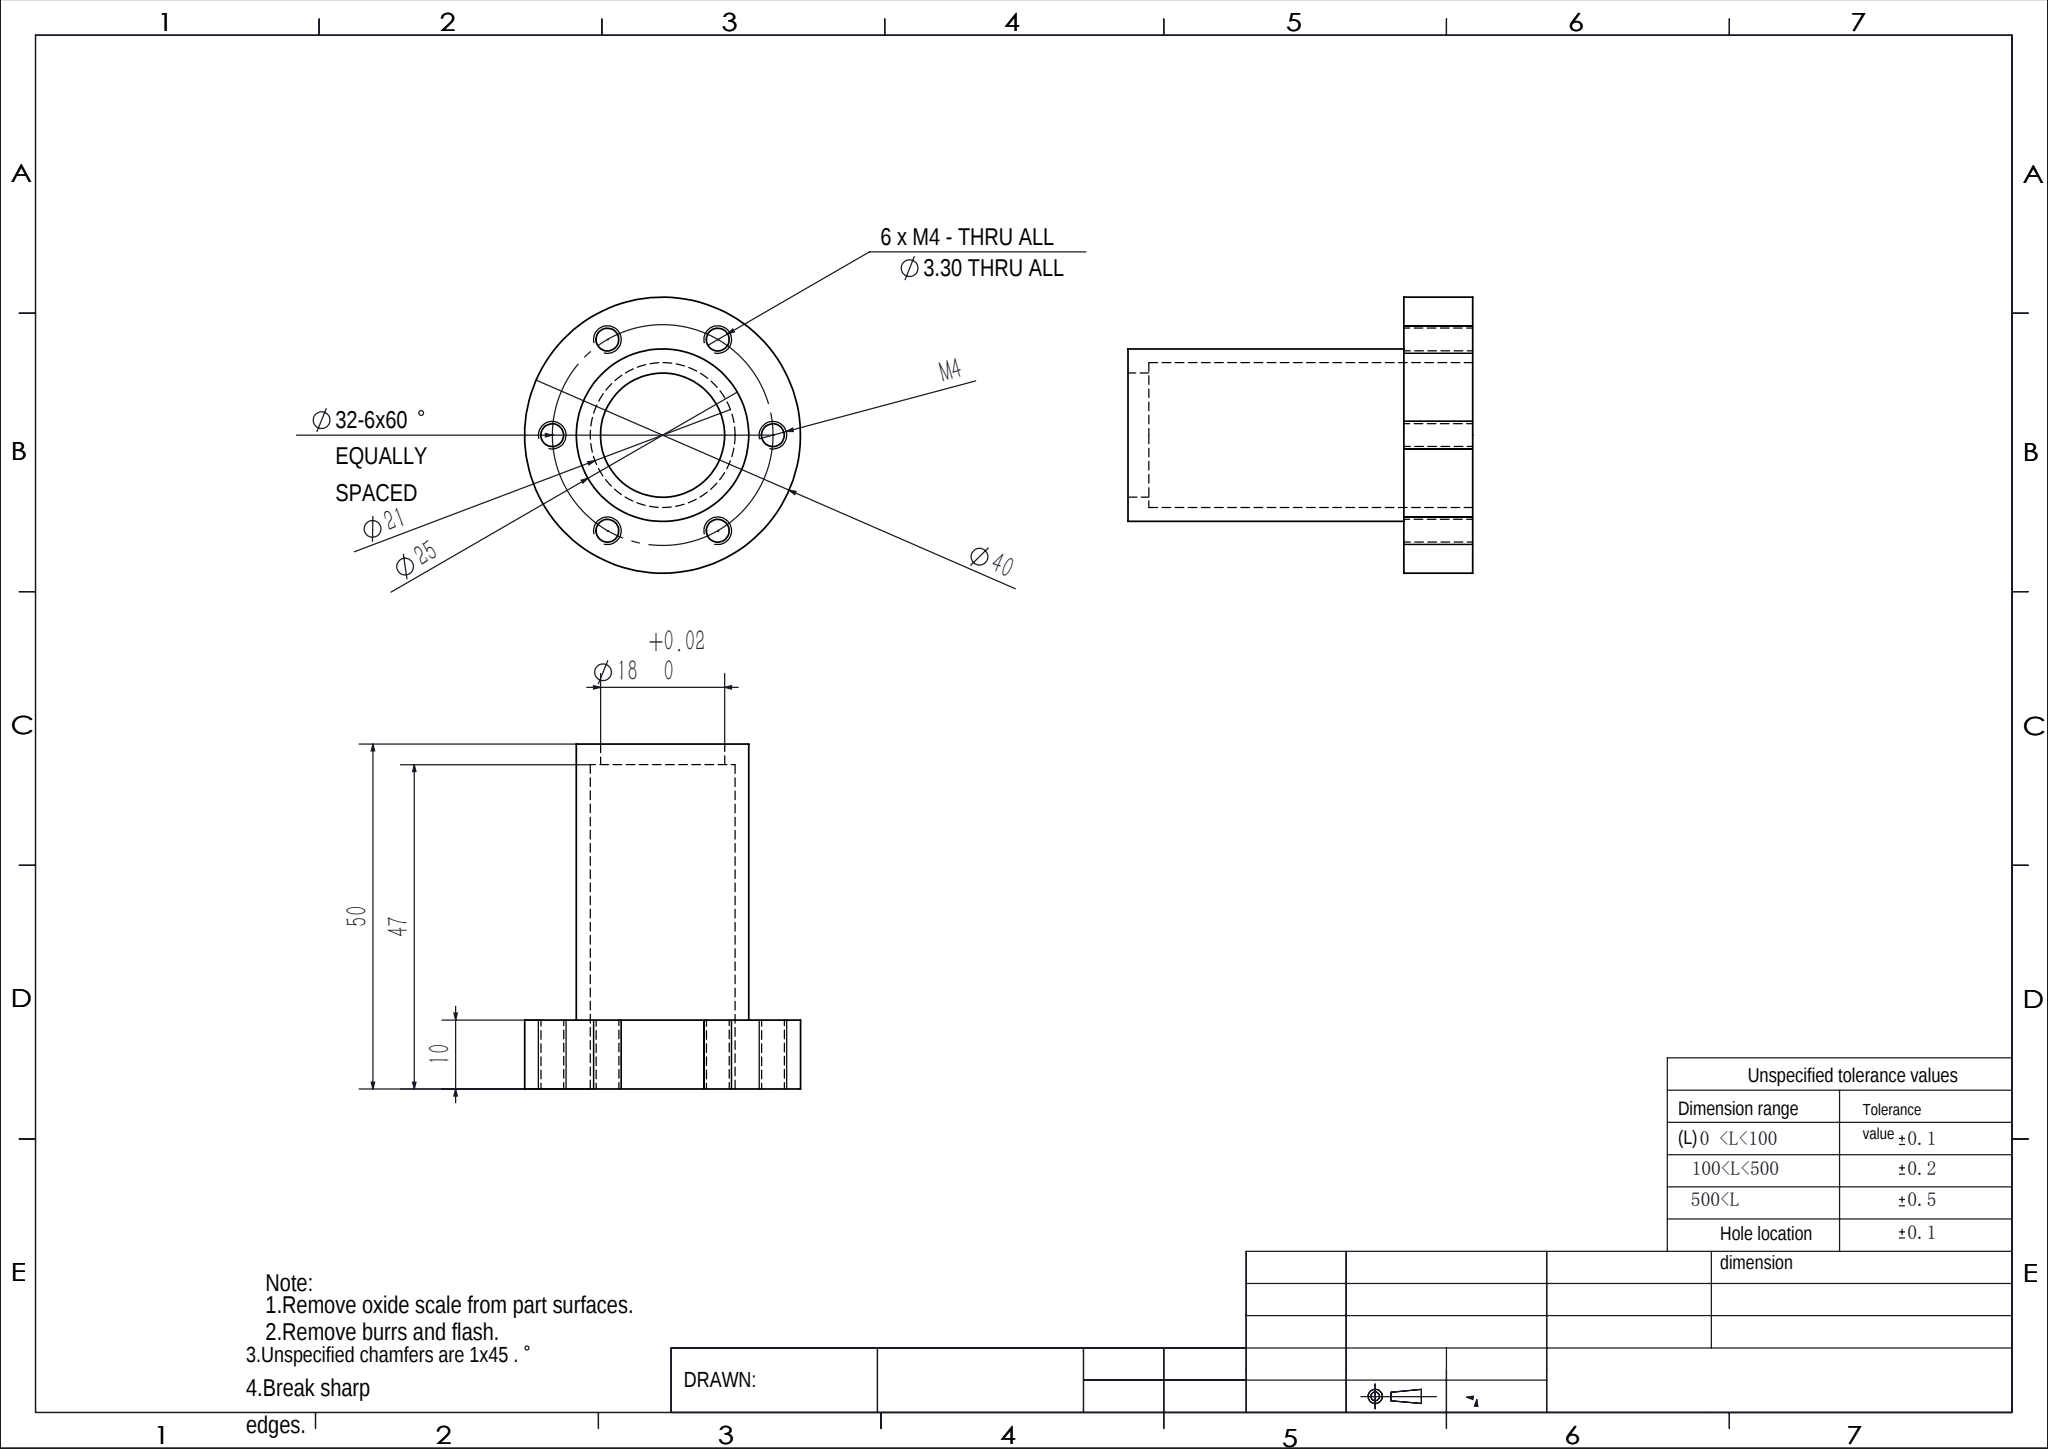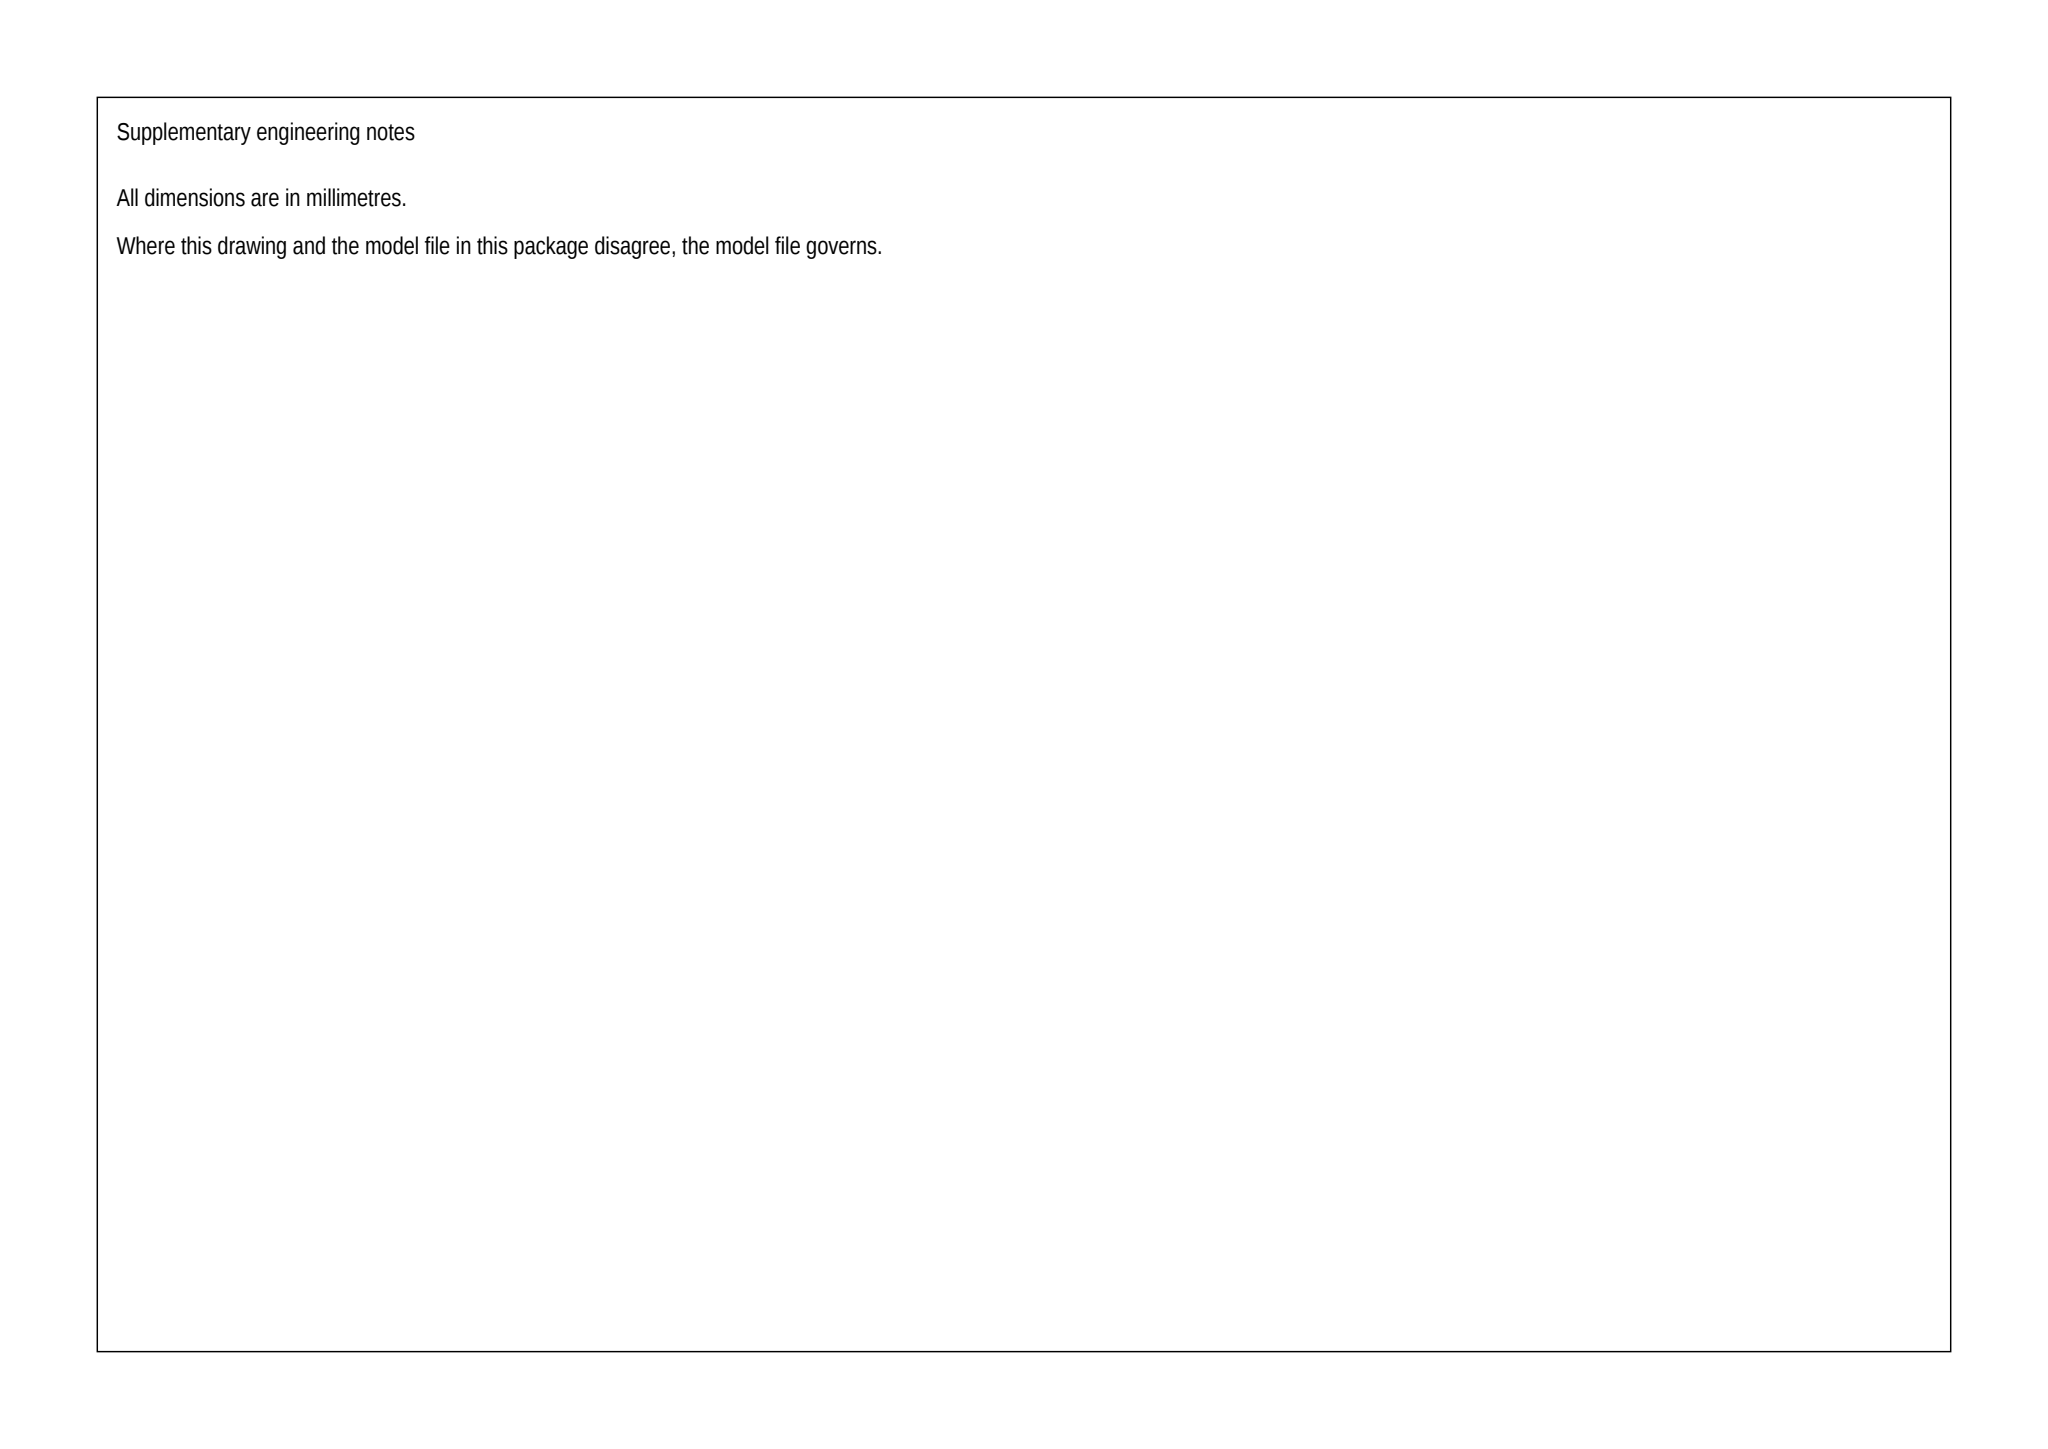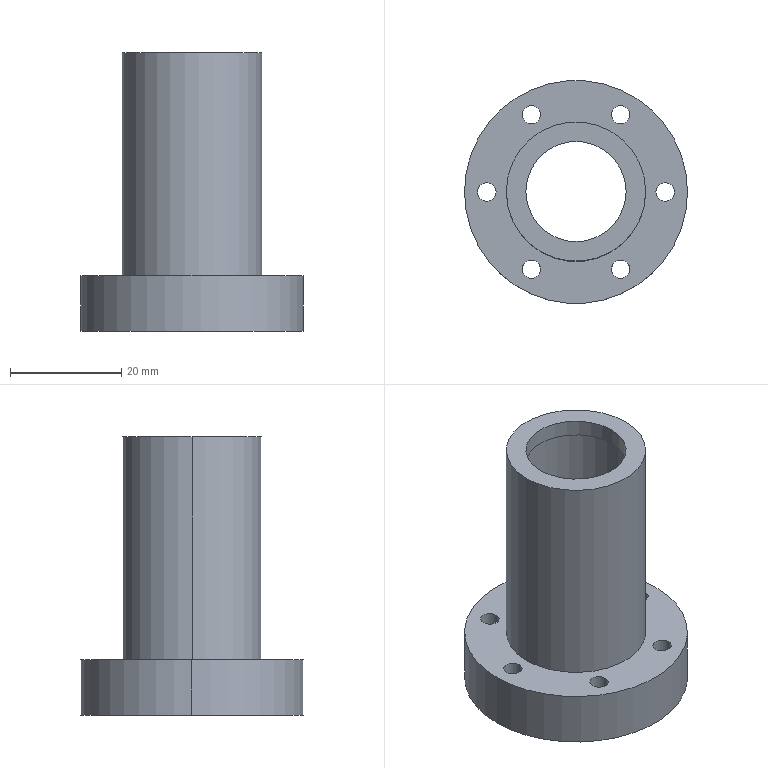Part | SolidWorks | mm | material 6061 | 1 solid | 24 faces | box 40 x 40 x 50 mm | volume 14646 mm3 | cylinder 20 | plane 4 | commonest cylinder face diameters 3.3 x12 25 x2 18 x2 40 x2 21 x2
Drawing notes:
UNSPECIFIED CHAMFERS 1 x 45 DEG; BLUNT SHARP CORNERS | from the solid: No inclined_planes/cones in STEP; garbled "1x454" = 1x45 deg chamfer note only
build123d program:
from build123d import *

# Parameters (mm, degrees)
SKETCH1_R           = 20
BOSS_EXTRUDE1_DEPTH = 50
SKETCH2_R           = 10.5
CUT_EXTRUDE1_DEPTH  = 58.446
BOSS_EXTRUDE2_START = -3
SKETCH3_R           = 10.5
SKETCH3_R_2         = 9
BOSS_EXTRUDE2_DEPTH = 3
CUT_EXTRUDE2_START  = -10
SKETCH4_R           = 23.5
SKETCH4_R_2         = 12.5
CUT_EXTRUDE2_DEPTH  = 48.446
M4_TAPPED_HOLE1_D   = 3.3


with BuildPart() as part:
    # Sketch1 → Boss-Extrude1 (new body)
    with BuildSketch(Plane.XY):
        Circle(SKETCH1_R)
    extrude(amount=BOSS_EXTRUDE1_DEPTH)

    # Sketch2 → Cut-Extrude1 (cut, through all)
    with BuildSketch(Plane(origin=(0, 0, 0), x_dir=(-1, 0, 0), z_dir=(0, 0, -1))):
        Circle(SKETCH2_R)
    extrude(amount=-CUT_EXTRUDE1_DEPTH, mode=Mode.SUBTRACT)

    # Sketch3 → Boss-Extrude2 (add)
    with BuildSketch(Plane.XY.offset(50).offset(BOSS_EXTRUDE2_START)):
        with Locations(Location((0, 0, 0), (0, 0, 180))):
            Circle(SKETCH3_R)
        Circle(SKETCH3_R_2, mode=Mode.SUBTRACT)
    extrude(amount=BOSS_EXTRUDE2_DEPTH)

    # Sketch4 → Cut-Extrude2 (cut, through all)
    with BuildSketch(Plane(origin=(0, 0, 0), x_dir=(-1, 0, 0), z_dir=(0, 0, -1)).offset(CUT_EXTRUDE2_START)):
        Circle(SKETCH4_R)
        Circle(SKETCH4_R_2, mode=Mode.SUBTRACT)
    extrude(amount=-CUT_EXTRUDE2_DEPTH, mode=Mode.SUBTRACT)

    # M4 Tapped Hole1 (through all)
    with Locations(Plane(origin=(0, 0, 0), x_dir=(-1, 0, 0), z_dir=(0, 0, -1))):
        with Locations((-16, 0), (-8, 13.856), (8, 13.856), (16, 0), (8, -13.856), (-8, -13.856), (0, 0)):
            Hole(M4_TAPPED_HOLE1_D / 2)


solid = part.part
STEP:
#1=CARTESIAN_POINT('',(17.65,0.,10.));
#2=VERTEX_POINT('',#1);
#3=CARTESIAN_POINT('',(14.35,0.,10.));
#4=VERTEX_POINT('',#3);
#5=CARTESIAN_POINT('',(16.,0.,10.));
#6=DIRECTION('',(0.,0.,-1.));
#7=DIRECTION('',(-1.,0.,0.));
#8=AXIS2_PLACEMENT_3D('',#5,#6,#7);
#9=CIRCLE('',#8,1.65);
#10=EDGE_CURVE('',#2,#4,#9,.T.);
#11=ORIENTED_EDGE('',*,*,#10,.F.);
#12=CARTESIAN_POINT('',(17.65,0.,-0.));
#13=VERTEX_POINT('',#12);
#14=CARTESIAN_POINT('',(17.65,0.,0.));
#15=DIRECTION('',(0.,0.,-1.));
#16=VECTOR('',#15,1000.);
#17=LINE('',#14,#16);
#18=EDGE_CURVE('',#2,#13,#17,.T.);
#19=ORIENTED_EDGE('',*,*,#18,.T.);
#20=CARTESIAN_POINT('',(14.35,0.,-0.));
#21=VERTEX_POINT('',#20);
#22=CARTESIAN_POINT('',(16.,0.,-0.));
#23=DIRECTION('',(0.,0.,-1.));
#24=DIRECTION('',(-1.,0.,0.));
#25=AXIS2_PLACEMENT_3D('',#22,#23,#24);
#26=CIRCLE('',#25,1.65);
#27=EDGE_CURVE('',#13,#21,#26,.T.);
#28=ORIENTED_EDGE('',*,*,#27,.T.);
#29=CARTESIAN_POINT('',(14.35,0.,0.));
#30=DIRECTION('',(0.,0.,-1.));
#31=VECTOR('',#30,1000.);
#32=LINE('',#29,#31);
#33=EDGE_CURVE('',#4,#21,#32,.T.);
#34=ORIENTED_EDGE('',*,*,#33,.F.);
#35=EDGE_LOOP('',(#11,#19,#28,#34));
#36=FACE_OUTER_BOUND('',#35,.T.);
#37=CARTESIAN_POINT('',(16.,0.,0.));
#38=DIRECTION('',(0.,0.,-1.));
#39=DIRECTION('',(-1.,0.,0.));
#40=AXIS2_PLACEMENT_3D('',#37,#38,#39);
#41=CYLINDRICAL_SURFACE('',#40,1.65);
#42=ADVANCED_FACE('',(#36),#41,.F.);
#43=CARTESIAN_POINT('',(9.65,13.856,10.));
#44=VERTEX_POINT('',#43);
#45=CARTESIAN_POINT('',(6.35,13.856,10.));
#46=VERTEX_POINT('',#45);
#47=CARTESIAN_POINT('',(8.,13.856,10.));
#48=DIRECTION('',(0.,0.,-1.));
#49=DIRECTION('',(-1.,0.,0.));
#50=AXIS2_PLACEMENT_3D('',#47,#48,#49);
#51=CIRCLE('',#50,1.65);
#52=EDGE_CURVE('',#44,#46,#51,.T.);
#53=ORIENTED_EDGE('',*,*,#52,.F.);
#54=CARTESIAN_POINT('',(9.65,13.856,-0.));
#55=VERTEX_POINT('',#54);
#56=CARTESIAN_POINT('',(9.65,13.856,0.));
#57=DIRECTION('',(0.,0.,-1.));
#58=VECTOR('',#57,1000.);
#59=LINE('',#56,#58);
#60=EDGE_CURVE('',#44,#55,#59,.T.);
#61=ORIENTED_EDGE('',*,*,#60,.T.);
#62=CARTESIAN_POINT('',(6.35,13.856,-0.));
#63=VERTEX_POINT('',#62);
#64=CARTESIAN_POINT('',(8.,13.856,-0.));
#65=DIRECTION('',(0.,0.,-1.));
#66=DIRECTION('',(-1.,0.,0.));
#67=AXIS2_PLACEMENT_3D('',#64,#65,#66);
#68=CIRCLE('',#67,1.65);
#69=EDGE_CURVE('',#55,#63,#68,.T.);
#70=ORIENTED_EDGE('',*,*,#69,.T.);
#71=CARTESIAN_POINT('',(6.35,13.856,0.));
#72=DIRECTION('',(0.,0.,-1.));
#73=VECTOR('',#72,1000.);
#74=LINE('',#71,#73);
#75=EDGE_CURVE('',#46,#63,#74,.T.);
#76=ORIENTED_EDGE('',*,*,#75,.F.);
#77=EDGE_LOOP('',(#53,#61,#70,#76));
#78=FACE_OUTER_BOUND('',#77,.T.);
#79=CARTESIAN_POINT('',(8.,13.856,0.));
#80=DIRECTION('',(0.,0.,-1.));
#81=DIRECTION('',(-1.,0.,0.));
#82=AXIS2_PLACEMENT_3D('',#79,#80,#81);
#83=CYLINDRICAL_SURFACE('',#82,1.65);
#84=ADVANCED_FACE('',(#78),#83,.F.);
#85=CARTESIAN_POINT('',(-6.35,13.856,10.));
#86=VERTEX_POINT('',#85);
#87=CARTESIAN_POINT('',(-9.65,13.856,10.));
#88=VERTEX_POINT('',#87);
#89=CARTESIAN_POINT('',(-8.,13.856,10.));
#90=DIRECTION('',(0.,0.,-1.));
#91=DIRECTION('',(-1.,0.,0.));
#92=AXIS2_PLACEMENT_3D('',#89,#90,#91);
#93=CIRCLE('',#92,1.65);
#94=EDGE_CURVE('',#86,#88,#93,.T.);
#95=ORIENTED_EDGE('',*,*,#94,.F.);
#96=CARTESIAN_POINT('',(-6.35,13.856,-0.));
#97=VERTEX_POINT('',#96);
#98=CARTESIAN_POINT('',(-6.35,13.856,0.));
#99=DIRECTION('',(0.,0.,-1.));
#100=VECTOR('',#99,1000.);
#101=LINE('',#98,#100);
#102=EDGE_CURVE('',#86,#97,#101,.T.);
#103=ORIENTED_EDGE('',*,*,#102,.T.);
#104=CARTESIAN_POINT('',(-9.65,13.856,-0.));
#105=VERTEX_POINT('',#104);
#106=CARTESIAN_POINT('',(-8.,13.856,-0.));
#107=DIRECTION('',(0.,0.,-1.));
#108=DIRECTION('',(-1.,0.,0.));
#109=AXIS2_PLACEMENT_3D('',#106,#107,#108);
#110=CIRCLE('',#109,1.65);
#111=EDGE_CURVE('',#97,#105,#110,.T.);
#112=ORIENTED_EDGE('',*,*,#111,.T.);
#113=CARTESIAN_POINT('',(-9.65,13.856,0.));
#114=DIRECTION('',(0.,0.,-1.));
#115=VECTOR('',#114,1000.);
#116=LINE('',#113,#115);
#117=EDGE_CURVE('',#88,#105,#116,.T.);
#118=ORIENTED_EDGE('',*,*,#117,.F.);
#119=EDGE_LOOP('',(#95,#103,#112,#118));
#120=FACE_OUTER_BOUND('',#119,.T.);
#121=CARTESIAN_POINT('',(-8.,13.856,0.));
#122=DIRECTION('',(0.,0.,-1.));
#123=DIRECTION('',(-1.,0.,0.));
#124=AXIS2_PLACEMENT_3D('',#121,#122,#123);
#125=CYLINDRICAL_SURFACE('',#124,1.65);
#126=ADVANCED_FACE('',(#120),#125,.F.);
#127=CARTESIAN_POINT('',(-14.35,-0.,10.));
#128=VERTEX_POINT('',#127);
#129=CARTESIAN_POINT('',(-17.65,-0.,10.));
#130=VERTEX_POINT('',#129);
#131=CARTESIAN_POINT('',(-16.,-0.,10.));
#132=DIRECTION('',(0.,0.,-1.));
#133=DIRECTION('',(-1.,0.,0.));
#134=AXIS2_PLACEMENT_3D('',#131,#132,#133);
#135=CIRCLE('',#134,1.65);
#136=EDGE_CURVE('',#128,#130,#135,.T.);
#137=ORIENTED_EDGE('',*,*,#136,.F.);
#138=CARTESIAN_POINT('',(-14.35,-0.,-0.));
#139=VERTEX_POINT('',#138);
#140=CARTESIAN_POINT('',(-14.35,-0.,0.));
#141=DIRECTION('',(0.,0.,-1.));
#142=VECTOR('',#141,1000.);
#143=LINE('',#140,#142);
#144=EDGE_CURVE('',#128,#139,#143,.T.);
#145=ORIENTED_EDGE('',*,*,#144,.T.);
#146=CARTESIAN_POINT('',(-17.65,-0.,-0.));
#147=VERTEX_POINT('',#146);
#148=CARTESIAN_POINT('',(-16.,-0.,-0.));
#149=DIRECTION('',(0.,0.,-1.));
#150=DIRECTION('',(-1.,0.,0.));
#151=AXIS2_PLACEMENT_3D('',#148,#149,#150);
#152=CIRCLE('',#151,1.65);
#153=EDGE_CURVE('',#139,#147,#152,.T.);
#154=ORIENTED_EDGE('',*,*,#153,.T.);
#155=CARTESIAN_POINT('',(-17.65,-0.,0.));
#156=DIRECTION('',(0.,0.,-1.));
#157=VECTOR('',#156,1000.);
#158=LINE('',#155,#157);
#159=EDGE_CURVE('',#130,#147,#158,.T.);
#160=ORIENTED_EDGE('',*,*,#159,.F.);
#161=EDGE_LOOP('',(#137,#145,#154,#160));
#162=FACE_OUTER_BOUND('',#161,.T.);
#163=CARTESIAN_POINT('',(-16.,-0.,0.));
#164=DIRECTION('',(0.,0.,-1.));
#165=DIRECTION('',(-1.,0.,0.));
#166=AXIS2_PLACEMENT_3D('',#163,#164,#165);
#167=CYLINDRICAL_SURFACE('',#166,1.65);
#168=ADVANCED_FACE('',(#162),#167,.F.);
#169=CARTESIAN_POINT('',(-6.35,-13.856,10.));
#170=VERTEX_POINT('',#169);
#171=CARTESIAN_POINT('',(-9.65,-13.856,10.));
#172=VERTEX_POINT('',#171);
#173=CARTESIAN_POINT('',(-8.,-13.856,10.));
#174=DIRECTION('',(0.,0.,-1.));
#175=DIRECTION('',(-1.,0.,0.));
#176=AXIS2_PLACEMENT_3D('',#173,#174,#175);
#177=CIRCLE('',#176,1.65);
#178=EDGE_CURVE('',#170,#172,#177,.T.);
#179=ORIENTED_EDGE('',*,*,#178,.F.);
#180=CARTESIAN_POINT('',(-6.35,-13.856,-0.));
#181=VERTEX_POINT('',#180);
#182=CARTESIAN_POINT('',(-6.35,-13.856,0.));
#183=DIRECTION('',(0.,0.,-1.));
#184=VECTOR('',#183,1000.);
#185=LINE('',#182,#184);
#186=EDGE_CURVE('',#170,#181,#185,.T.);
#187=ORIENTED_EDGE('',*,*,#186,.T.);
#188=CARTESIAN_POINT('',(-9.65,-13.856,-0.));
#189=VERTEX_POINT('',#188);
#190=CARTESIAN_POINT('',(-8.,-13.856,-0.));
#191=DIRECTION('',(0.,0.,-1.));
#192=DIRECTION('',(-1.,0.,0.));
#193=AXIS2_PLACEMENT_3D('',#190,#191,#192);
#194=CIRCLE('',#193,1.65);
#195=EDGE_CURVE('',#181,#189,#194,.T.);
#196=ORIENTED_EDGE('',*,*,#195,.T.);
#197=CARTESIAN_POINT('',(-9.65,-13.856,0.));
#198=DIRECTION('',(0.,0.,-1.));
#199=VECTOR('',#198,1000.);
#200=LINE('',#197,#199);
#201=EDGE_CURVE('',#172,#189,#200,.T.);
#202=ORIENTED_EDGE('',*,*,#201,.F.);
#203=EDGE_LOOP('',(#179,#187,#196,#202));
#204=FACE_OUTER_BOUND('',#203,.T.);
#205=CARTESIAN_POINT('',(-8.,-13.856,0.));
#206=DIRECTION('',(0.,0.,-1.));
#207=DIRECTION('',(-1.,0.,0.));
#208=AXIS2_PLACEMENT_3D('',#205,#206,#207);
#209=CYLINDRICAL_SURFACE('',#208,1.65);
#210=ADVANCED_FACE('',(#204),#209,.F.);
#211=CARTESIAN_POINT('',(9.65,-13.856,10.));
#212=VERTEX_POINT('',#211);
#213=CARTESIAN_POINT('',(6.35,-13.856,10.));
#214=VERTEX_POINT('',#213);
#215=CARTESIAN_POINT('',(8.,-13.856,10.));
#216=DIRECTION('',(0.,0.,-1.));
#217=DIRECTION('',(-1.,0.,0.));
#218=AXIS2_PLACEMENT_3D('',#215,#216,#217);
#219=CIRCLE('',#218,1.65);
#220=EDGE_CURVE('',#212,#214,#219,.T.);
#221=ORIENTED_EDGE('',*,*,#220,.F.);
#222=CARTESIAN_POINT('',(9.65,-13.856,-0.));
#223=VERTEX_POINT('',#222);
#224=CARTESIAN_POINT('',(9.65,-13.856,0.));
#225=DIRECTION('',(0.,0.,-1.));
#226=VECTOR('',#225,1000.);
#227=LINE('',#224,#226);
#228=EDGE_CURVE('',#212,#223,#227,.T.);
#229=ORIENTED_EDGE('',*,*,#228,.T.);
#230=CARTESIAN_POINT('',(6.35,-13.856,-0.));
#231=VERTEX_POINT('',#230);
#232=CARTESIAN_POINT('',(8.,-13.856,-0.));
#233=DIRECTION('',(0.,0.,-1.));
#234=DIRECTION('',(-1.,0.,0.));
#235=AXIS2_PLACEMENT_3D('',#232,#233,#234);
#236=CIRCLE('',#235,1.65);
#237=EDGE_CURVE('',#223,#231,#236,.T.);
#238=ORIENTED_EDGE('',*,*,#237,.T.);
#239=CARTESIAN_POINT('',(6.35,-13.856,0.));
#240=DIRECTION('',(0.,0.,-1.));
#241=VECTOR('',#240,1000.);
#242=LINE('',#239,#241);
#243=EDGE_CURVE('',#214,#231,#242,.T.);
#244=ORIENTED_EDGE('',*,*,#243,.F.);
#245=EDGE_LOOP('',(#221,#229,#238,#244));
#246=FACE_OUTER_BOUND('',#245,.T.);
#247=CARTESIAN_POINT('',(8.,-13.856,0.));
#248=DIRECTION('',(0.,0.,-1.));
#249=DIRECTION('',(-1.,0.,0.));
#250=AXIS2_PLACEMENT_3D('',#247,#248,#249);
#251=CYLINDRICAL_SURFACE('',#250,1.65);
#252=ADVANCED_FACE('',(#246),#251,.F.);
#253=CARTESIAN_POINT('',(-12.5,0.,50.));
#254=VERTEX_POINT('',#253);
#255=CARTESIAN_POINT('',(12.5,0.,50.));
#256=VERTEX_POINT('',#255);
#257=CARTESIAN_POINT('',(0.,0.,50.));
#258=DIRECTION('',(0.,0.,-1.));
#259=DIRECTION('',(-1.,0.,0.));
#260=AXIS2_PLACEMENT_3D('',#257,#258,#259);
#261=CIRCLE('',#260,12.5);
#262=EDGE_CURVE('',#254,#256,#261,.T.);
#263=ORIENTED_EDGE('',*,*,#262,.T.);
#264=CARTESIAN_POINT('',(12.5,0.,10.));
#265=VERTEX_POINT('',#264);
#266=CARTESIAN_POINT('',(12.5,0.,50.));
#267=DIRECTION('',(0.,0.,-1.));
#268=VECTOR('',#267,1000.);
#269=LINE('',#266,#268);
#270=EDGE_CURVE('',#256,#265,#269,.T.);
#271=ORIENTED_EDGE('',*,*,#270,.T.);
#272=CARTESIAN_POINT('',(-12.5,0.,10.));
#273=VERTEX_POINT('',#272);
#274=CARTESIAN_POINT('',(0.,0.,10.));
#275=DIRECTION('',(0.,0.,-1.));
#276=DIRECTION('',(-1.,0.,0.));
#277=AXIS2_PLACEMENT_3D('',#274,#275,#276);
#278=CIRCLE('',#277,12.5);
#279=EDGE_CURVE('',#273,#265,#278,.T.);
#280=ORIENTED_EDGE('',*,*,#279,.F.);
#281=CARTESIAN_POINT('',(-12.5,0.,50.));
#282=DIRECTION('',(0.,0.,-1.));
#283=VECTOR('',#282,1000.);
#284=LINE('',#281,#283);
#285=EDGE_CURVE('',#254,#273,#284,.T.);
#286=ORIENTED_EDGE('',*,*,#285,.F.);
#287=EDGE_LOOP('',(#263,#271,#280,#286));
#288=FACE_OUTER_BOUND('',#287,.T.);
#289=CARTESIAN_POINT('',(0.,0.,50.));
#290=DIRECTION('',(0.,0.,-1.));
#291=DIRECTION('',(-1.,0.,0.));
#292=AXIS2_PLACEMENT_3D('',#289,#290,#291);
#293=CYLINDRICAL_SURFACE('',#292,12.5);
#294=ADVANCED_FACE('',(#288),#293,.T.);
#295=CARTESIAN_POINT('',(-9.,-0.,47.));
#296=VERTEX_POINT('',#295);
#297=CARTESIAN_POINT('',(9.,-0.,47.));
#298=VERTEX_POINT('',#297);
#299=CARTESIAN_POINT('',(-0.,-0.,47.));
#300=DIRECTION('',(0.,0.,1.));
#301=DIRECTION('',(1.,0.,0.));
#302=AXIS2_PLACEMENT_3D('',#299,#300,#301);
#303=CIRCLE('',#302,9.);
#304=EDGE_CURVE('',#296,#298,#303,.T.);
#305=ORIENTED_EDGE('',*,*,#304,.F.);
#306=CARTESIAN_POINT('',(-9.,-0.,50.));
#307=VERTEX_POINT('',#306);
#308=CARTESIAN_POINT('',(-9.,-0.,47.));
#309=DIRECTION('',(0.,0.,1.));
#310=VECTOR('',#309,1000.);
#311=LINE('',#308,#310);
#312=EDGE_CURVE('',#296,#307,#311,.T.);
#313=ORIENTED_EDGE('',*,*,#312,.T.);
#314=CARTESIAN_POINT('',(9.,-0.,50.));
#315=VERTEX_POINT('',#314);
#316=CARTESIAN_POINT('',(-0.,-0.,50.));
#317=DIRECTION('',(0.,0.,1.));
#318=DIRECTION('',(1.,0.,0.));
#319=AXIS2_PLACEMENT_3D('',#316,#317,#318);
#320=CIRCLE('',#319,9.);
#321=EDGE_CURVE('',#307,#315,#320,.T.);
#322=ORIENTED_EDGE('',*,*,#321,.T.);
#323=CARTESIAN_POINT('',(9.,-0.,47.));
#324=DIRECTION('',(0.,0.,1.));
#325=VECTOR('',#324,1000.);
#326=LINE('',#323,#325);
#327=EDGE_CURVE('',#298,#315,#326,.T.);
#328=ORIENTED_EDGE('',*,*,#327,.F.);
#329=EDGE_LOOP('',(#305,#313,#322,#328));
#330=FACE_OUTER_BOUND('',#329,.T.);
#331=CARTESIAN_POINT('',(-0.,-0.,47.));
#332=DIRECTION('',(0.,0.,1.));
#333=DIRECTION('',(1.,0.,0.));
#334=AXIS2_PLACEMENT_3D('',#331,#332,#333);
#335=CYLINDRICAL_SURFACE('',#334,9.);
#336=ADVANCED_FACE('',(#330),#335,.F.);
#337=CARTESIAN_POINT('',(-20.,0.,10.));
#338=VERTEX_POINT('',#337);
#339=CARTESIAN_POINT('',(20.,0.,10.));
#340=VERTEX_POINT('',#339);
#341=CARTESIAN_POINT('',(0.,0.,10.));
#342=DIRECTION('',(0.,0.,-1.));
#343=DIRECTION('',(-1.,0.,0.));
#344=AXIS2_PLACEMENT_3D('',#341,#342,#343);
#345=CIRCLE('',#344,20.);
#346=EDGE_CURVE('',#338,#340,#345,.T.);
#347=ORIENTED_EDGE('',*,*,#346,.T.);
#348=CARTESIAN_POINT('',(20.,0.,0.));
#349=VERTEX_POINT('',#348);
#350=CARTESIAN_POINT('',(20.,0.,50.));
#351=DIRECTION('',(0.,0.,-1.));
#352=VECTOR('',#351,1000.);
#353=LINE('',#350,#352);
#354=EDGE_CURVE('',#340,#349,#353,.T.);
#355=ORIENTED_EDGE('',*,*,#354,.T.);
#356=CARTESIAN_POINT('',(-20.,0.,0.));
#357=VERTEX_POINT('',#356);
#358=CARTESIAN_POINT('',(0.,0.,0.));
#359=DIRECTION('',(0.,0.,1.));
#360=DIRECTION('',(1.,0.,0.));
#361=AXIS2_PLACEMENT_3D('',#358,#359,#360);
#362=CIRCLE('',#361,20.);
#363=EDGE_CURVE('',#349,#357,#362,.T.);
#364=ORIENTED_EDGE('',*,*,#363,.T.);
#365=CARTESIAN_POINT('',(-20.,0.,50.));
#366=DIRECTION('',(0.,0.,-1.));
#367=VECTOR('',#366,1000.);
#368=LINE('',#365,#367);
#369=EDGE_CURVE('',#338,#357,#368,.T.);
#370=ORIENTED_EDGE('',*,*,#369,.F.);
#371=EDGE_LOOP('',(#347,#355,#364,#370));
#372=FACE_OUTER_BOUND('',#371,.T.);
#373=CARTESIAN_POINT('',(0.,0.,50.));
#374=DIRECTION('',(0.,0.,-1.));
#375=DIRECTION('',(-1.,0.,0.));
#376=AXIS2_PLACEMENT_3D('',#373,#374,#375);
#377=CYLINDRICAL_SURFACE('',#376,20.);
#378=ADVANCED_FACE('',(#372),#377,.T.);
#379=CARTESIAN_POINT('',(10.5,0.,47.));
#380=VERTEX_POINT('',#379);
#381=CARTESIAN_POINT('',(-10.5,0.,47.));
#382=VERTEX_POINT('',#381);
#383=CARTESIAN_POINT('',(0.,0.,47.));
#384=DIRECTION('',(0.,0.,-1.));
#385=DIRECTION('',(1.,0.,0.));
#386=AXIS2_PLACEMENT_3D('',#383,#384,#385);
#387=CIRCLE('',#386,10.5);
#388=EDGE_CURVE('',#380,#382,#387,.T.);
#389=ORIENTED_EDGE('',*,*,#388,.F.);
#390=CARTESIAN_POINT('',(10.5,0.,0.));
#391=VERTEX_POINT('',#390);
#392=CARTESIAN_POINT('',(10.5,0.,50.));
#393=DIRECTION('',(0.,0.,-1.));
#394=VECTOR('',#393,1000.);
#395=LINE('',#392,#394);
#396=EDGE_CURVE('',#380,#391,#395,.T.);
#397=ORIENTED_EDGE('',*,*,#396,.T.);
#398=CARTESIAN_POINT('',(-10.5,0.,0.));
#399=VERTEX_POINT('',#398);
#400=CARTESIAN_POINT('',(0.,0.,0.));
#401=DIRECTION('',(0.,0.,-1.));
#402=DIRECTION('',(-1.,0.,0.));
#403=AXIS2_PLACEMENT_3D('',#400,#401,#402);
#404=CIRCLE('',#403,10.5);
#405=EDGE_CURVE('',#391,#399,#404,.T.);
#406=ORIENTED_EDGE('',*,*,#405,.T.);
#407=CARTESIAN_POINT('',(-10.5,0.,50.));
#408=DIRECTION('',(0.,0.,-1.));
#409=VECTOR('',#408,1000.);
#410=LINE('',#407,#409);
#411=EDGE_CURVE('',#382,#399,#410,.T.);
#412=ORIENTED_EDGE('',*,*,#411,.F.);
#413=EDGE_LOOP('',(#389,#397,#406,#412));
#414=FACE_OUTER_BOUND('',#413,.T.);
#415=CARTESIAN_POINT('',(0.,0.,50.));
#416=DIRECTION('',(0.,0.,-1.));
#417=DIRECTION('',(-1.,0.,0.));
#418=AXIS2_PLACEMENT_3D('',#415,#416,#417);
#419=CYLINDRICAL_SURFACE('',#418,10.5);
#420=ADVANCED_FACE('',(#414),#419,.F.);
#421=CARTESIAN_POINT('',(-0.,-0.,50.));
#422=DIRECTION('',(0.,0.,1.));
#423=DIRECTION('',(1.,0.,0.));
#424=AXIS2_PLACEMENT_3D('',#421,#422,#423);
#425=CIRCLE('',#424,9.);
#426=EDGE_CURVE('',#315,#307,#425,.T.);
#427=ORIENTED_EDGE('',*,*,#426,.F.);
#428=ORIENTED_EDGE('',*,*,#321,.F.);
#429=EDGE_LOOP('',(#427,#428));
#430=FACE_BOUND('',#429,.T.);
#431=ORIENTED_EDGE('',*,*,#262,.F.);
#432=CARTESIAN_POINT('',(0.,0.,50.));
#433=DIRECTION('',(0.,0.,-1.));
#434=DIRECTION('',(-1.,0.,0.));
#435=AXIS2_PLACEMENT_3D('',#432,#433,#434);
#436=CIRCLE('',#435,12.5);
#437=EDGE_CURVE('',#256,#254,#436,.T.);
#438=ORIENTED_EDGE('',*,*,#437,.F.);
#439=EDGE_LOOP('',(#431,#438));
#440=FACE_OUTER_BOUND('',#439,.T.);
#441=CARTESIAN_POINT('',(0.,0.,50.));
#442=DIRECTION('',(0.,0.,1.));
#443=DIRECTION('',(1.,0.,0.));
#444=AXIS2_PLACEMENT_3D('',#441,#442,#443);
#445=PLANE('',#444);
#446=ADVANCED_FACE('',(#430,#440),#445,.T.);
#447=ORIENTED_EDGE('',*,*,#396,.F.);
#448=CARTESIAN_POINT('',(0.,0.,47.));
#449=DIRECTION('',(0.,0.,-1.));
#450=DIRECTION('',(1.,0.,0.));
#451=AXIS2_PLACEMENT_3D('',#448,#449,#450);
#452=CIRCLE('',#451,10.5);
#453=EDGE_CURVE('',#382,#380,#452,.T.);
#454=ORIENTED_EDGE('',*,*,#453,.F.);
#455=ORIENTED_EDGE('',*,*,#411,.T.);
#456=CARTESIAN_POINT('',(0.,0.,0.));
#457=DIRECTION('',(0.,0.,-1.));
#458=DIRECTION('',(-1.,0.,0.));
#459=AXIS2_PLACEMENT_3D('',#456,#457,#458);
#460=CIRCLE('',#459,10.5);
#461=EDGE_CURVE('',#399,#391,#460,.T.);
#462=ORIENTED_EDGE('',*,*,#461,.T.);
#463=EDGE_LOOP('',(#447,#454,#455,#462));
#464=FACE_OUTER_BOUND('',#463,.T.);
#465=CARTESIAN_POINT('',(0.,0.,50.));
#466=DIRECTION('',(0.,0.,-1.));
#467=DIRECTION('',(-1.,0.,0.));
#468=AXIS2_PLACEMENT_3D('',#465,#466,#467);
#469=CYLINDRICAL_SURFACE('',#468,10.5);
#470=ADVANCED_FACE('',(#464),#469,.F.);
#471=ORIENTED_EDGE('',*,*,#354,.F.);
#472=CARTESIAN_POINT('',(0.,0.,10.));
#473=DIRECTION('',(0.,0.,-1.));
#474=DIRECTION('',(-1.,0.,0.));
#475=AXIS2_PLACEMENT_3D('',#472,#473,#474);
#476=CIRCLE('',#475,20.);
#477=EDGE_CURVE('',#340,#338,#476,.T.);
#478=ORIENTED_EDGE('',*,*,#477,.T.);
#479=ORIENTED_EDGE('',*,*,#369,.T.);
#480=CARTESIAN_POINT('',(0.,0.,0.));
#481=DIRECTION('',(0.,0.,1.));
#482=DIRECTION('',(1.,0.,0.));
#483=AXIS2_PLACEMENT_3D('',#480,#481,#482);
#484=CIRCLE('',#483,20.);
#485=EDGE_CURVE('',#357,#349,#484,.T.);
#486=ORIENTED_EDGE('',*,*,#485,.T.);
#487=EDGE_LOOP('',(#471,#478,#479,#486));
#488=FACE_OUTER_BOUND('',#487,.T.);
#489=CARTESIAN_POINT('',(0.,0.,50.));
#490=DIRECTION('',(0.,0.,-1.));
#491=DIRECTION('',(-1.,0.,0.));
#492=AXIS2_PLACEMENT_3D('',#489,#490,#491);
#493=CYLINDRICAL_SURFACE('',#492,20.);
#494=ADVANCED_FACE('',(#488),#493,.T.);
#495=CARTESIAN_POINT('',(16.,0.,-0.));
#496=DIRECTION('',(0.,0.,-1.));
#497=DIRECTION('',(-1.,0.,0.));
#498=AXIS2_PLACEMENT_3D('',#495,#496,#497);
#499=CIRCLE('',#498,1.65);
#500=EDGE_CURVE('',#21,#13,#499,.T.);
#501=ORIENTED_EDGE('',*,*,#500,.F.);
#502=ORIENTED_EDGE('',*,*,#27,.F.);
#503=EDGE_LOOP('',(#501,#502));
#504=FACE_BOUND('',#503,.T.);
#505=CARTESIAN_POINT('',(8.,13.856,-0.));
#506=DIRECTION('',(0.,0.,-1.));
#507=DIRECTION('',(-1.,0.,0.));
#508=AXIS2_PLACEMENT_3D('',#505,#506,#507);
#509=CIRCLE('',#508,1.65);
#510=EDGE_CURVE('',#63,#55,#509,.T.);
#511=ORIENTED_EDGE('',*,*,#510,.F.);
#512=ORIENTED_EDGE('',*,*,#69,.F.);
#513=EDGE_LOOP('',(#511,#512));
#514=FACE_BOUND('',#513,.T.);
#515=CARTESIAN_POINT('',(-8.,13.856,-0.));
#516=DIRECTION('',(0.,0.,-1.));
#517=DIRECTION('',(-1.,0.,0.));
#518=AXIS2_PLACEMENT_3D('',#515,#516,#517);
#519=CIRCLE('',#518,1.65);
#520=EDGE_CURVE('',#105,#97,#519,.T.);
#521=ORIENTED_EDGE('',*,*,#520,.F.);
#522=ORIENTED_EDGE('',*,*,#111,.F.);
#523=EDGE_LOOP('',(#521,#522));
#524=FACE_BOUND('',#523,.T.);
#525=CARTESIAN_POINT('',(-16.,-0.,-0.));
#526=DIRECTION('',(0.,0.,-1.));
#527=DIRECTION('',(-1.,0.,0.));
#528=AXIS2_PLACEMENT_3D('',#525,#526,#527);
#529=CIRCLE('',#528,1.65);
#530=EDGE_CURVE('',#147,#139,#529,.T.);
#531=ORIENTED_EDGE('',*,*,#530,.F.);
#532=ORIENTED_EDGE('',*,*,#153,.F.);
#533=EDGE_LOOP('',(#531,#532));
#534=FACE_BOUND('',#533,.T.);
#535=CARTESIAN_POINT('',(-8.,-13.856,-0.));
#536=DIRECTION('',(0.,0.,-1.));
#537=DIRECTION('',(-1.,0.,0.));
#538=AXIS2_PLACEMENT_3D('',#535,#536,#537);
#539=CIRCLE('',#538,1.65);
#540=EDGE_CURVE('',#189,#181,#539,.T.);
#541=ORIENTED_EDGE('',*,*,#540,.F.);
#542=ORIENTED_EDGE('',*,*,#195,.F.);
#543=EDGE_LOOP('',(#541,#542));
#544=FACE_BOUND('',#543,.T.);
#545=CARTESIAN_POINT('',(8.,-13.856,-0.));
#546=DIRECTION('',(0.,0.,-1.));
#547=DIRECTION('',(-1.,0.,0.));
#548=AXIS2_PLACEMENT_3D('',#545,#546,#547);
#549=CIRCLE('',#548,1.65);
#550=EDGE_CURVE('',#231,#223,#549,.T.);
#551=ORIENTED_EDGE('',*,*,#550,.F.);
#552=ORIENTED_EDGE('',*,*,#237,.F.);
#553=EDGE_LOOP('',(#551,#552));
#554=FACE_BOUND('',#553,.T.);
#555=ORIENTED_EDGE('',*,*,#461,.F.);
#556=ORIENTED_EDGE('',*,*,#405,.F.);
#557=EDGE_LOOP('',(#555,#556));
#558=FACE_BOUND('',#557,.T.);
#559=ORIENTED_EDGE('',*,*,#485,.F.);
#560=ORIENTED_EDGE('',*,*,#363,.F.);
#561=EDGE_LOOP('',(#559,#560));
#562=FACE_OUTER_BOUND('',#561,.T.);
#563=CARTESIAN_POINT('',(0.,0.,0.));
#564=DIRECTION('',(0.,0.,1.));
#565=DIRECTION('',(1.,0.,0.));
#566=AXIS2_PLACEMENT_3D('',#563,#564,#565);
#567=PLANE('',#566);
#568=ADVANCED_FACE('',(#504,#514,#524,#534,#544,#554,#558,#562),#567,.F.);
#569=CARTESIAN_POINT('',(-0.,-0.,47.));
#570=DIRECTION('',(0.,0.,1.));
#571=DIRECTION('',(1.,0.,0.));
#572=AXIS2_PLACEMENT_3D('',#569,#570,#571);
#573=CIRCLE('',#572,9.);
#574=EDGE_CURVE('',#298,#296,#573,.T.);
#575=ORIENTED_EDGE('',*,*,#574,.T.);
#576=ORIENTED_EDGE('',*,*,#304,.T.);
#577=EDGE_LOOP('',(#575,#576));
#578=FACE_BOUND('',#577,.T.);
#579=ORIENTED_EDGE('',*,*,#453,.T.);
#580=ORIENTED_EDGE('',*,*,#388,.T.);
#581=EDGE_LOOP('',(#579,#580));
#582=FACE_OUTER_BOUND('',#581,.T.);
#583=CARTESIAN_POINT('',(-0.,-0.,47.));
#584=DIRECTION('',(0.,0.,1.));
#585=DIRECTION('',(1.,0.,0.));
#586=AXIS2_PLACEMENT_3D('',#583,#584,#585);
#587=PLANE('',#586);
#588=ADVANCED_FACE('',(#578,#582),#587,.F.);
#589=ORIENTED_EDGE('',*,*,#312,.F.);
#590=ORIENTED_EDGE('',*,*,#574,.F.);
#591=ORIENTED_EDGE('',*,*,#327,.T.);
#592=ORIENTED_EDGE('',*,*,#426,.T.);
#593=EDGE_LOOP('',(#589,#590,#591,#592));
#594=FACE_OUTER_BOUND('',#593,.T.);
#595=CARTESIAN_POINT('',(-0.,-0.,47.));
#596=DIRECTION('',(0.,0.,1.));
#597=DIRECTION('',(1.,0.,0.));
#598=AXIS2_PLACEMENT_3D('',#595,#596,#597);
#599=CYLINDRICAL_SURFACE('',#598,9.);
#600=ADVANCED_FACE('',(#594),#599,.F.);
#601=CARTESIAN_POINT('',(16.,0.,10.));
#602=DIRECTION('',(0.,0.,-1.));
#603=DIRECTION('',(-1.,0.,0.));
#604=AXIS2_PLACEMENT_3D('',#601,#602,#603);
#605=CIRCLE('',#604,1.65);
#606=EDGE_CURVE('',#4,#2,#605,.T.);
#607=ORIENTED_EDGE('',*,*,#606,.T.);
#608=ORIENTED_EDGE('',*,*,#10,.T.);
#609=EDGE_LOOP('',(#607,#608));
#610=FACE_BOUND('',#609,.T.);
#611=CARTESIAN_POINT('',(8.,13.856,10.));
#612=DIRECTION('',(0.,0.,-1.));
#613=DIRECTION('',(-1.,0.,0.));
#614=AXIS2_PLACEMENT_3D('',#611,#612,#613);
#615=CIRCLE('',#614,1.65);
#616=EDGE_CURVE('',#46,#44,#615,.T.);
#617=ORIENTED_EDGE('',*,*,#616,.T.);
#618=ORIENTED_EDGE('',*,*,#52,.T.);
#619=EDGE_LOOP('',(#617,#618));
#620=FACE_BOUND('',#619,.T.);
#621=CARTESIAN_POINT('',(-8.,13.856,10.));
#622=DIRECTION('',(0.,0.,-1.));
#623=DIRECTION('',(-1.,0.,0.));
#624=AXIS2_PLACEMENT_3D('',#621,#622,#623);
#625=CIRCLE('',#624,1.65);
#626=EDGE_CURVE('',#88,#86,#625,.T.);
#627=ORIENTED_EDGE('',*,*,#626,.T.);
#628=ORIENTED_EDGE('',*,*,#94,.T.);
#629=EDGE_LOOP('',(#627,#628));
#630=FACE_BOUND('',#629,.T.);
#631=CARTESIAN_POINT('',(-16.,-0.,10.));
#632=DIRECTION('',(0.,0.,-1.));
#633=DIRECTION('',(-1.,0.,0.));
#634=AXIS2_PLACEMENT_3D('',#631,#632,#633);
#635=CIRCLE('',#634,1.65);
#636=EDGE_CURVE('',#130,#128,#635,.T.);
#637=ORIENTED_EDGE('',*,*,#636,.T.);
#638=ORIENTED_EDGE('',*,*,#136,.T.);
#639=EDGE_LOOP('',(#637,#638));
#640=FACE_BOUND('',#639,.T.);
#641=CARTESIAN_POINT('',(-8.,-13.856,10.));
#642=DIRECTION('',(0.,0.,-1.));
#643=DIRECTION('',(-1.,0.,0.));
#644=AXIS2_PLACEMENT_3D('',#641,#642,#643);
#645=CIRCLE('',#644,1.65);
#646=EDGE_CURVE('',#172,#170,#645,.T.);
#647=ORIENTED_EDGE('',*,*,#646,.T.);
#648=ORIENTED_EDGE('',*,*,#178,.T.);
#649=EDGE_LOOP('',(#647,#648));
#650=FACE_BOUND('',#649,.T.);
#651=CARTESIAN_POINT('',(8.,-13.856,10.));
#652=DIRECTION('',(0.,0.,-1.));
#653=DIRECTION('',(-1.,0.,0.));
#654=AXIS2_PLACEMENT_3D('',#651,#652,#653);
#655=CIRCLE('',#654,1.65);
#656=EDGE_CURVE('',#214,#212,#655,.T.);
#657=ORIENTED_EDGE('',*,*,#656,.T.);
#658=ORIENTED_EDGE('',*,*,#220,.T.);
#659=EDGE_LOOP('',(#657,#658));
#660=FACE_BOUND('',#659,.T.);
#661=ORIENTED_EDGE('',*,*,#279,.T.);
#662=CARTESIAN_POINT('',(0.,0.,10.));
#663=DIRECTION('',(0.,0.,-1.));
#664=DIRECTION('',(-1.,0.,0.));
#665=AXIS2_PLACEMENT_3D('',#662,#663,#664);
#666=CIRCLE('',#665,12.5);
#667=EDGE_CURVE('',#265,#273,#666,.T.);
#668=ORIENTED_EDGE('',*,*,#667,.T.);
#669=EDGE_LOOP('',(#661,#668));
#670=FACE_BOUND('',#669,.T.);
#671=ORIENTED_EDGE('',*,*,#346,.F.);
#672=ORIENTED_EDGE('',*,*,#477,.F.);
#673=EDGE_LOOP('',(#671,#672));
#674=FACE_OUTER_BOUND('',#673,.T.);
#675=CARTESIAN_POINT('',(0.,0.,10.));
#676=DIRECTION('',(0.,0.,-1.));
#677=DIRECTION('',(-1.,0.,0.));
#678=AXIS2_PLACEMENT_3D('',#675,#676,#677);
#679=PLANE('',#678);
#680=ADVANCED_FACE('',(#610,#620,#630,#640,#650,#660,#670,#674),#679,.F.);
#681=ORIENTED_EDGE('',*,*,#270,.F.);
#682=ORIENTED_EDGE('',*,*,#437,.T.);
#683=ORIENTED_EDGE('',*,*,#285,.T.);
#684=ORIENTED_EDGE('',*,*,#667,.F.);
#685=EDGE_LOOP('',(#681,#682,#683,#684));
#686=FACE_OUTER_BOUND('',#685,.T.);
#687=CARTESIAN_POINT('',(0.,0.,50.));
#688=DIRECTION('',(0.,0.,-1.));
#689=DIRECTION('',(-1.,0.,0.));
#690=AXIS2_PLACEMENT_3D('',#687,#688,#689);
#691=CYLINDRICAL_SURFACE('',#690,12.5);
#692=ADVANCED_FACE('',(#686),#691,.T.);
#693=ORIENTED_EDGE('',*,*,#228,.F.);
#694=ORIENTED_EDGE('',*,*,#656,.F.);
#695=ORIENTED_EDGE('',*,*,#243,.T.);
#696=ORIENTED_EDGE('',*,*,#550,.T.);
#697=EDGE_LOOP('',(#693,#694,#695,#696));
#698=FACE_OUTER_BOUND('',#697,.T.);
#699=CARTESIAN_POINT('',(8.,-13.856,0.));
#700=DIRECTION('',(0.,0.,-1.));
#701=DIRECTION('',(-1.,0.,0.));
#702=AXIS2_PLACEMENT_3D('',#699,#700,#701);
#703=CYLINDRICAL_SURFACE('',#702,1.65);
#704=ADVANCED_FACE('',(#698),#703,.F.);
#705=ORIENTED_EDGE('',*,*,#186,.F.);
#706=ORIENTED_EDGE('',*,*,#646,.F.);
#707=ORIENTED_EDGE('',*,*,#201,.T.);
#708=ORIENTED_EDGE('',*,*,#540,.T.);
#709=EDGE_LOOP('',(#705,#706,#707,#708));
#710=FACE_OUTER_BOUND('',#709,.T.);
#711=CARTESIAN_POINT('',(-8.,-13.856,0.));
#712=DIRECTION('',(0.,0.,-1.));
#713=DIRECTION('',(-1.,0.,0.));
#714=AXIS2_PLACEMENT_3D('',#711,#712,#713);
#715=CYLINDRICAL_SURFACE('',#714,1.65);
#716=ADVANCED_FACE('',(#710),#715,.F.);
#717=ORIENTED_EDGE('',*,*,#144,.F.);
#718=ORIENTED_EDGE('',*,*,#636,.F.);
#719=ORIENTED_EDGE('',*,*,#159,.T.);
#720=ORIENTED_EDGE('',*,*,#530,.T.);
#721=EDGE_LOOP('',(#717,#718,#719,#720));
#722=FACE_OUTER_BOUND('',#721,.T.);
#723=CARTESIAN_POINT('',(-16.,-0.,0.));
#724=DIRECTION('',(0.,0.,-1.));
#725=DIRECTION('',(-1.,0.,0.));
#726=AXIS2_PLACEMENT_3D('',#723,#724,#725);
#727=CYLINDRICAL_SURFACE('',#726,1.65);
#728=ADVANCED_FACE('',(#722),#727,.F.);
#729=ORIENTED_EDGE('',*,*,#102,.F.);
#730=ORIENTED_EDGE('',*,*,#626,.F.);
#731=ORIENTED_EDGE('',*,*,#117,.T.);
#732=ORIENTED_EDGE('',*,*,#520,.T.);
#733=EDGE_LOOP('',(#729,#730,#731,#732));
#734=FACE_OUTER_BOUND('',#733,.T.);
#735=CARTESIAN_POINT('',(-8.,13.856,0.));
#736=DIRECTION('',(0.,0.,-1.));
#737=DIRECTION('',(-1.,0.,0.));
#738=AXIS2_PLACEMENT_3D('',#735,#736,#737);
#739=CYLINDRICAL_SURFACE('',#738,1.65);
#740=ADVANCED_FACE('',(#734),#739,.F.);
#741=ORIENTED_EDGE('',*,*,#60,.F.);
#742=ORIENTED_EDGE('',*,*,#616,.F.);
#743=ORIENTED_EDGE('',*,*,#75,.T.);
#744=ORIENTED_EDGE('',*,*,#510,.T.);
#745=EDGE_LOOP('',(#741,#742,#743,#744));
#746=FACE_OUTER_BOUND('',#745,.T.);
#747=CARTESIAN_POINT('',(8.,13.856,0.));
#748=DIRECTION('',(0.,0.,-1.));
#749=DIRECTION('',(-1.,0.,0.));
#750=AXIS2_PLACEMENT_3D('',#747,#748,#749);
#751=CYLINDRICAL_SURFACE('',#750,1.65);
#752=ADVANCED_FACE('',(#746),#751,.F.);
#753=ORIENTED_EDGE('',*,*,#18,.F.);
#754=ORIENTED_EDGE('',*,*,#606,.F.);
#755=ORIENTED_EDGE('',*,*,#33,.T.);
#756=ORIENTED_EDGE('',*,*,#500,.T.);
#757=EDGE_LOOP('',(#753,#754,#755,#756));
#758=FACE_OUTER_BOUND('',#757,.T.);
#759=CARTESIAN_POINT('',(16.,0.,0.));
#760=DIRECTION('',(0.,0.,-1.));
#761=DIRECTION('',(-1.,0.,0.));
#762=AXIS2_PLACEMENT_3D('',#759,#760,#761);
#763=CYLINDRICAL_SURFACE('',#762,1.65);
#764=ADVANCED_FACE('',(#758),#763,.F.);
#765=CLOSED_SHELL('',(#42,#84,#126,#168,#210,#252,#294,#336,#378,#420,#446,#470,#494,#568,#588,#600,#680,#692,#704,#716,#728,#740,#752,#764));
#766=MANIFOLD_SOLID_BREP('',#765);
#767=CARTESIAN_POINT('',(0.,0.,0.));
#768=DIRECTION('',(0.,0.,1.));
#769=DIRECTION('',(1.,0.,0.));
#770=AXIS2_PLACEMENT_3D('',#767,#768,#769);
#771=(LENGTH_UNIT()NAMED_UNIT(*)SI_UNIT(.MILLI.,.METRE.));
#772=UNCERTAINTY_MEASURE_WITH_UNIT(LENGTH_MEASURE(0.00001),#771,'','');
#773=(NAMED_UNIT(*)PLANE_ANGLE_UNIT()SI_UNIT($,.RADIAN.));
#774=(NAMED_UNIT(*)SI_UNIT($,.STERADIAN.)SOLID_ANGLE_UNIT());
#775=(GEOMETRIC_REPRESENTATION_CONTEXT(3)GLOBAL_UNCERTAINTY_ASSIGNED_CONTEXT((#772))GLOBAL_UNIT_ASSIGNED_CONTEXT((#771,#773,#774))REPRESENTATION_CONTEXT('',''));
#776=ADVANCED_BREP_SHAPE_REPRESENTATION('',(#766,#770),#775);